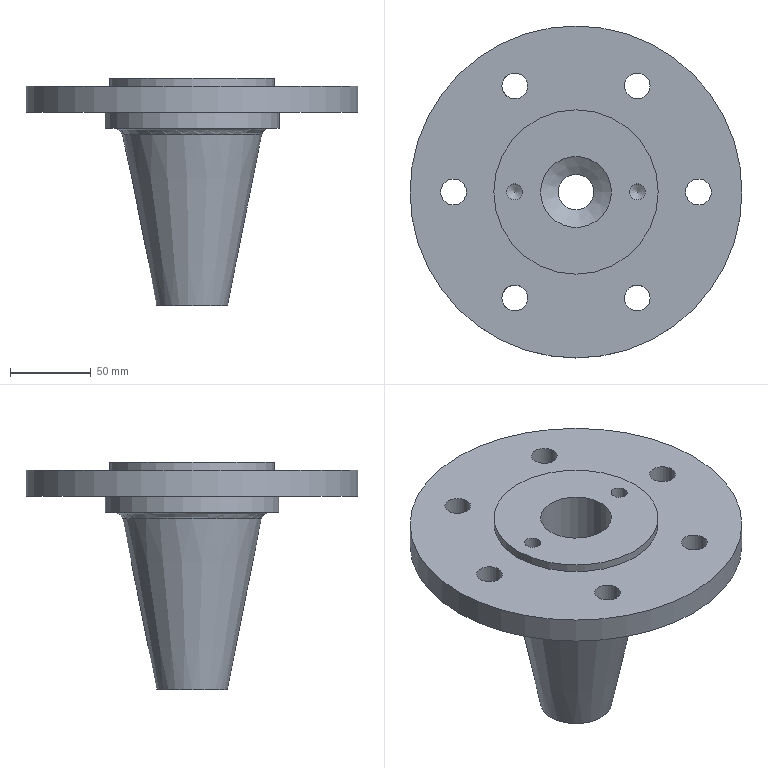Component | NX | 02__COVER__2 | 1 solid | 27 faces | volume 915664 mm3 | cylinder 15 | cone 6 | plane 5 | torus 1 | commonest cylinder face diameters 16 x6 10 x2 206 x1 102 x1 44 x1 22 x1 32 x1 25 x1